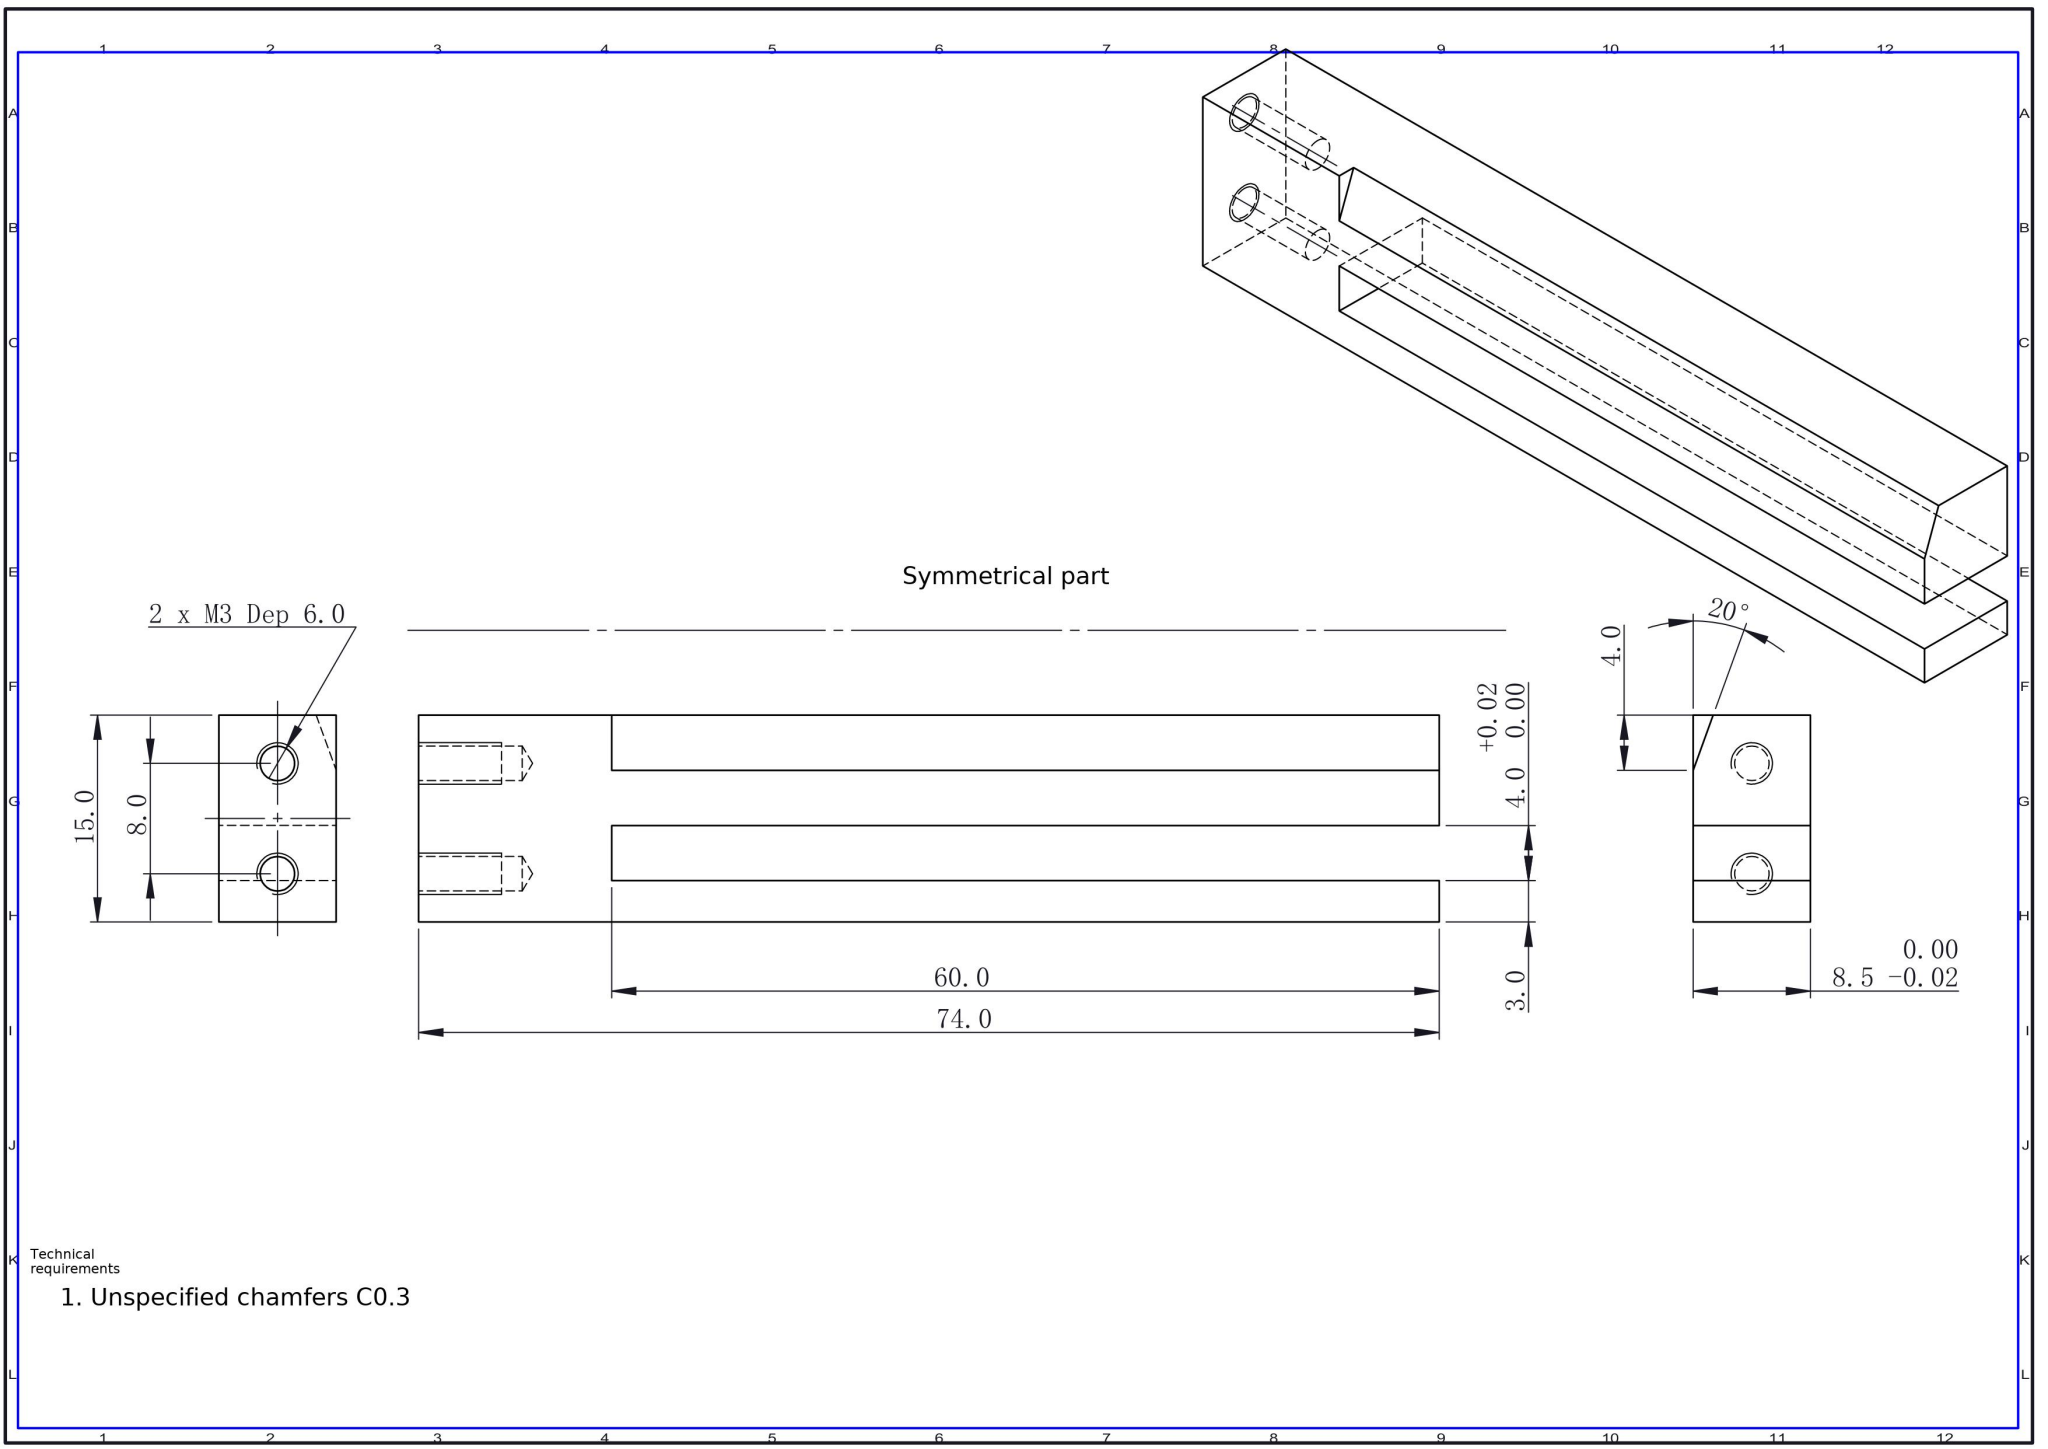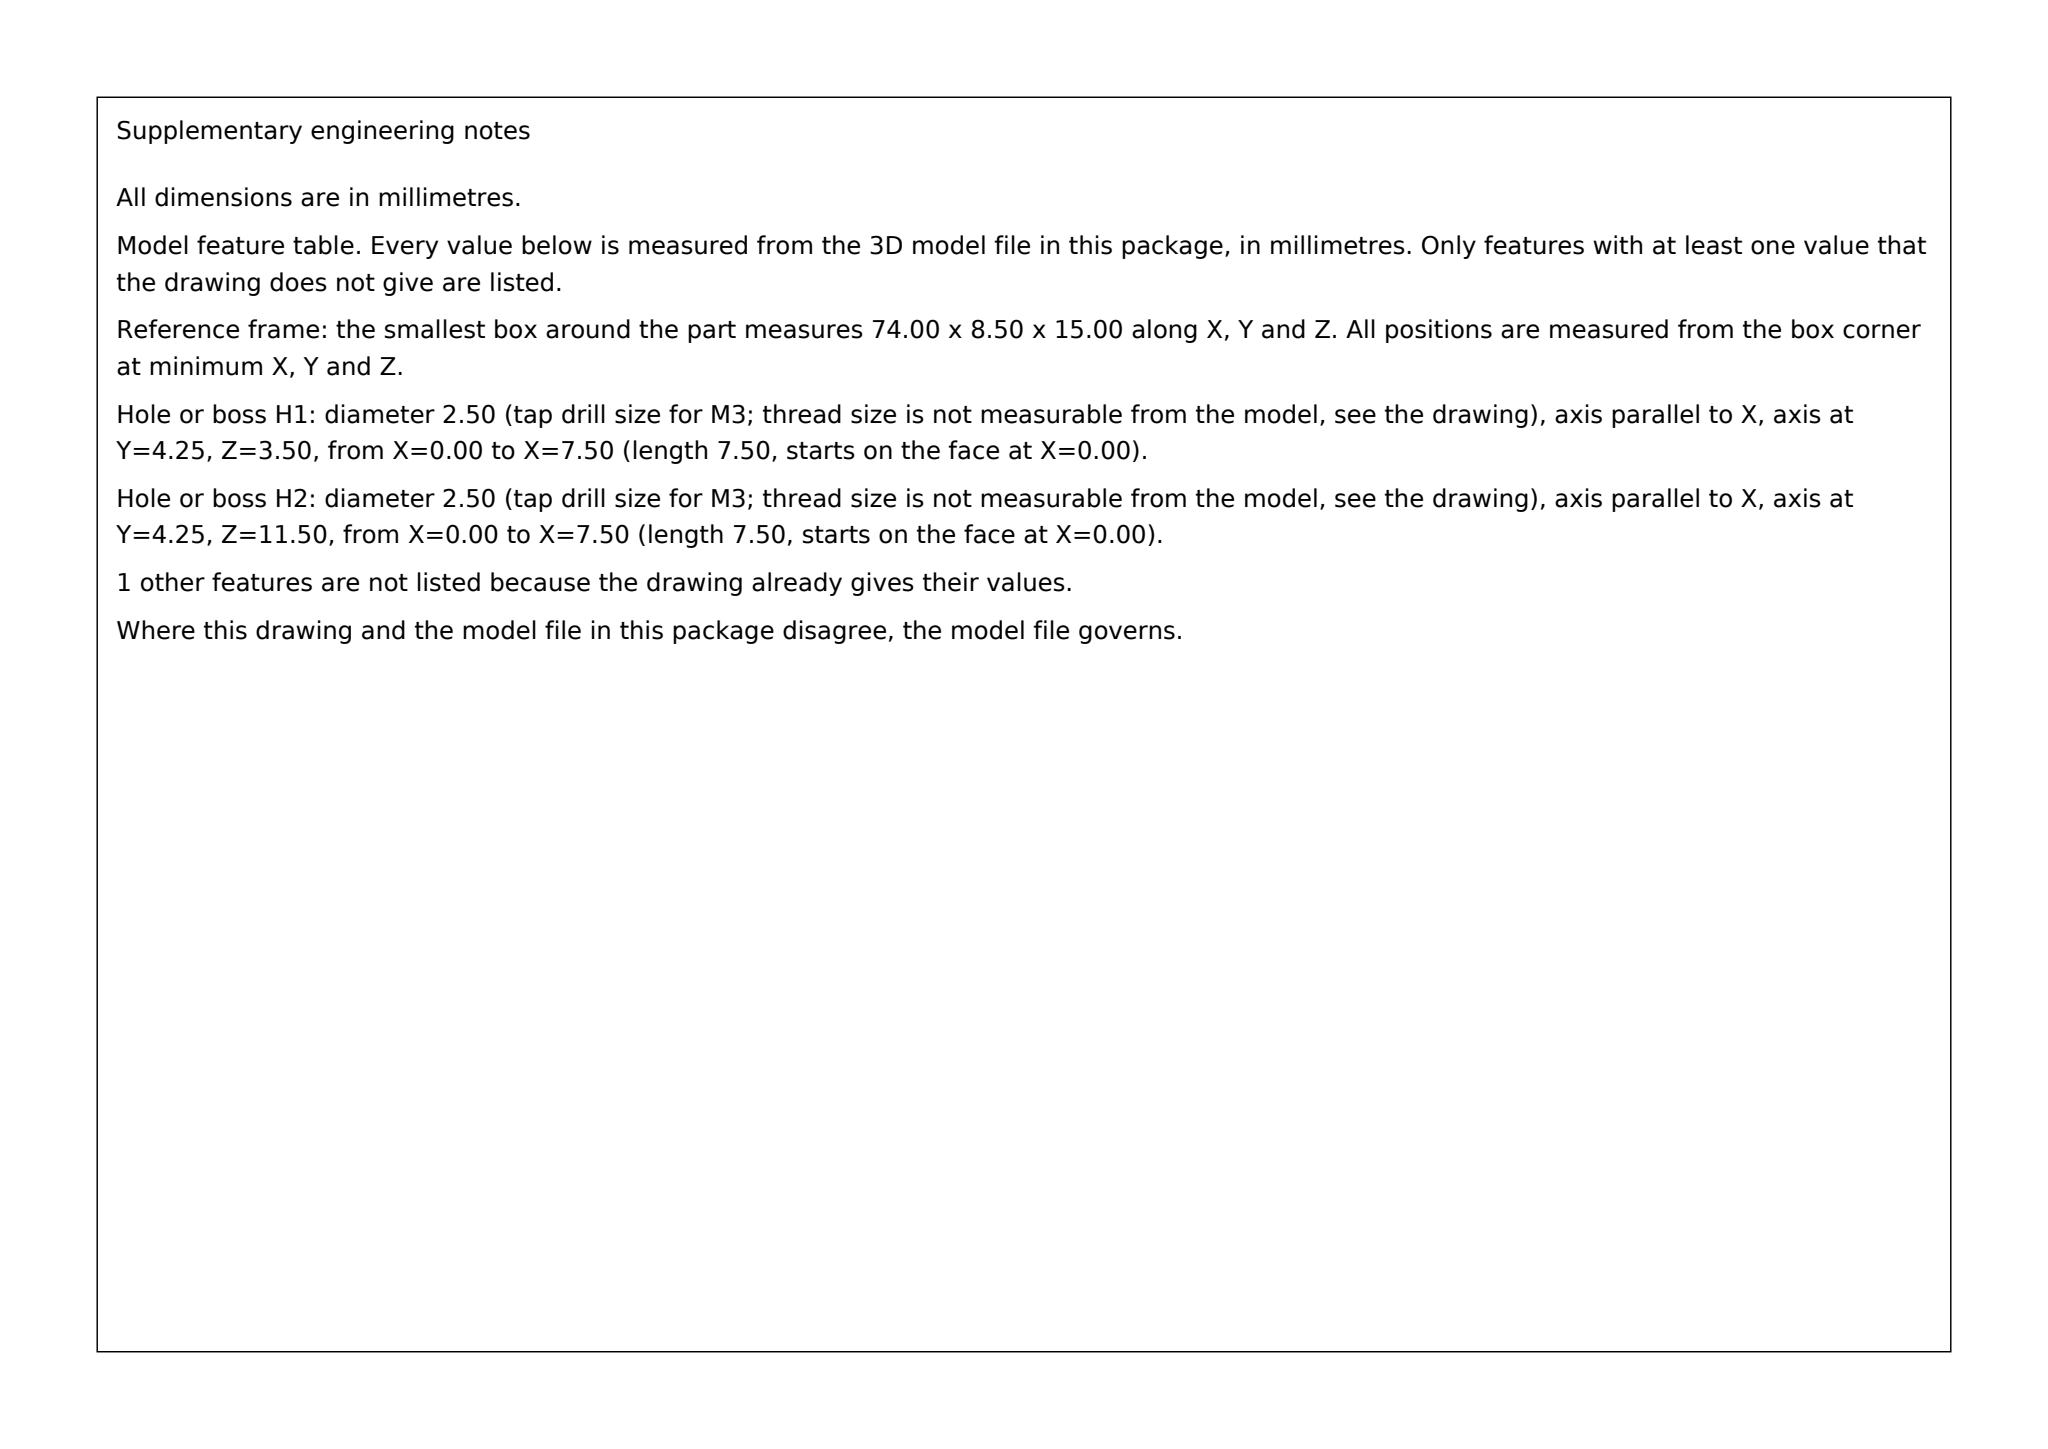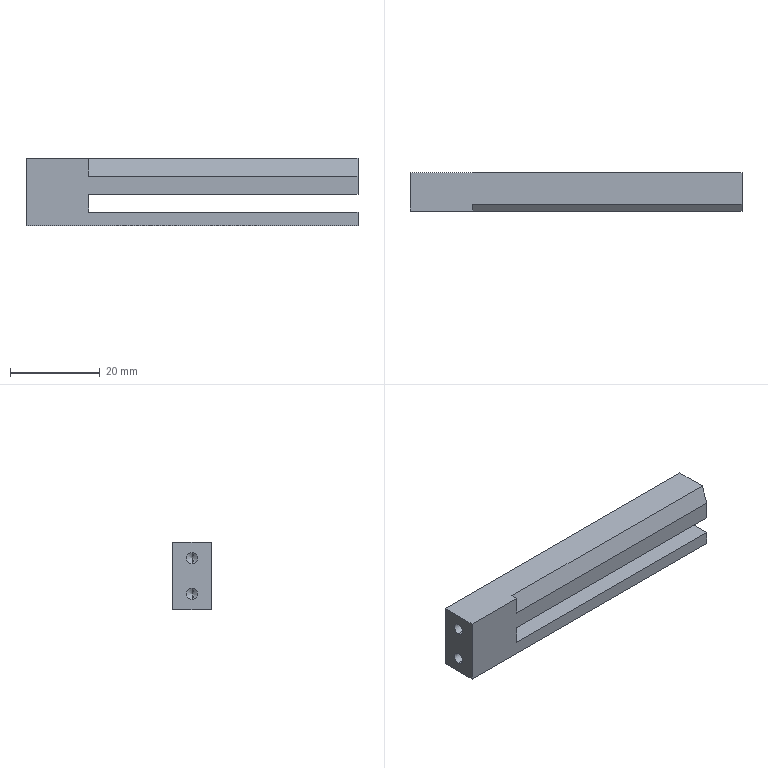Part | SolidWorks | mm | 1 solid | 20 faces | box 74 x 8.5 x 15 mm | volume 7144 mm3 | plane 12 | cylinder 4 | cone 4 | commonest cylinder face diameters 2.5 x4
build123d program:
from build123d import *

# Parameters (mm, degrees)
SKETCH1_W             = 74
SKETCH1_H             = 8.5
BOSS_EXTRUDE1_DEPTH   = 15
SKETCH4_W             = 60
SKETCH4_H             = 4
CUT_EXTRUDE1_DEPTH    = 76.982
M3_TAPPED_HOLE1_D     = 2.5
M3_TAPPED_HOLE1_DEPTH = 7.5
M3_TAPPED_HOLE1_TIP   = 0.7511
CUT_EXTRUDE2_DEPTH    = 60


with BuildPart() as part:
    # Sketch1 → Boss-Extrude1 (new body)
    with BuildSketch(Plane.XY):
        with Locations((37, 4.25)):
            Rectangle(SKETCH1_W, SKETCH1_H)
    extrude(amount=BOSS_EXTRUDE1_DEPTH)

    # Sketch4 → Cut-Extrude1 (cut, through all)
    with BuildSketch(Plane.XZ):
        with Locations((44, 5)):
            Rectangle(SKETCH4_W, SKETCH4_H)
    extrude(amount=-CUT_EXTRUDE1_DEPTH, mode=Mode.SUBTRACT)

    # M3 Tapped Hole1
    with Locations(Plane.ZY):
        with Locations((11.5, 4.25), (3.5, 4.25)):
            Hole(M3_TAPPED_HOLE1_D / 2, depth=M3_TAPPED_HOLE1_DEPTH)
            with Locations((0, 0, -(M3_TAPPED_HOLE1_DEPTH + M3_TAPPED_HOLE1_TIP / 2))):  # 118° drill point
                Cone(0, M3_TAPPED_HOLE1_D / 2, M3_TAPPED_HOLE1_TIP, mode=Mode.SUBTRACT)

    # Sketch7 → Cut-Extrude2 (cut)
    with BuildSketch(Plane(origin=(74, 0, 0), x_dir=(0, 0, -1), z_dir=(1, 0, 0))):
        Polygon((-15, 1.456), (-11, 0), (-15, 0), align=None)
    extrude(amount=-CUT_EXTRUDE2_DEPTH, mode=Mode.SUBTRACT)


solid = part.part
STEP:
#1=CARTESIAN_POINT('',(7.5,4.25,10.25));
#2=VERTEX_POINT('',#1);
#3=CARTESIAN_POINT('',(7.5,4.25,12.75));
#4=VERTEX_POINT('',#3);
#5=CARTESIAN_POINT('',(7.5,4.25,11.5));
#6=DIRECTION('',(-1.,0.,0.));
#7=DIRECTION('',(0.,0.,1.));
#8=AXIS2_PLACEMENT_3D('',#5,#6,#7);
#9=CIRCLE('',#8,1.25);
#10=EDGE_CURVE('',#2,#4,#9,.T.);
#11=ORIENTED_EDGE('',*,*,#10,.F.);
#12=CARTESIAN_POINT('',(-0.,4.25,10.25));
#13=VERTEX_POINT('',#12);
#14=CARTESIAN_POINT('',(0.,4.25,10.25));
#15=DIRECTION('',(-1.,0.,0.));
#16=VECTOR('',#15,1000.);
#17=LINE('',#14,#16);
#18=EDGE_CURVE('',#2,#13,#17,.T.);
#19=ORIENTED_EDGE('',*,*,#18,.T.);
#20=CARTESIAN_POINT('',(-0.,4.25,12.75));
#21=VERTEX_POINT('',#20);
#22=CARTESIAN_POINT('',(-0.,4.25,11.5));
#23=DIRECTION('',(-1.,0.,0.));
#24=DIRECTION('',(0.,0.,1.));
#25=AXIS2_PLACEMENT_3D('',#22,#23,#24);
#26=CIRCLE('',#25,1.25);
#27=EDGE_CURVE('',#13,#21,#26,.T.);
#28=ORIENTED_EDGE('',*,*,#27,.T.);
#29=CARTESIAN_POINT('',(0.,4.25,12.75));
#30=DIRECTION('',(-1.,0.,0.));
#31=VECTOR('',#30,1000.);
#32=LINE('',#29,#31);
#33=EDGE_CURVE('',#4,#21,#32,.T.);
#34=ORIENTED_EDGE('',*,*,#33,.F.);
#35=EDGE_LOOP('',(#11,#19,#28,#34));
#36=FACE_OUTER_BOUND('',#35,.T.);
#37=CARTESIAN_POINT('',(0.,4.25,11.5));
#38=DIRECTION('',(-1.,0.,0.));
#39=DIRECTION('',(0.,0.,1.));
#40=AXIS2_PLACEMENT_3D('',#37,#38,#39);
#41=CYLINDRICAL_SURFACE('',#40,1.25);
#42=ADVANCED_FACE('',(#36),#41,.F.);
#43=CARTESIAN_POINT('',(8.251,4.25,11.5));
#44=VERTEX_POINT('',#43);
#45=CARTESIAN_POINT('',(7.5,4.25,12.75));
#46=DIRECTION('',(-0.515,0.,0.8572));
#47=VECTOR('',#46,1000.);
#48=LINE('',#45,#47);
#49=EDGE_CURVE('',#44,#4,#48,.T.);
#50=ORIENTED_EDGE('',*,*,#49,.F.);
#51=CARTESIAN_POINT('',(7.5,4.25,10.25));
#52=DIRECTION('',(-0.515,0.,-0.8572));
#53=VECTOR('',#52,1000.);
#54=LINE('',#51,#53);
#55=EDGE_CURVE('',#44,#2,#54,.T.);
#56=ORIENTED_EDGE('',*,*,#55,.T.);
#57=ORIENTED_EDGE('',*,*,#10,.T.);
#58=EDGE_LOOP('',(#50,#56,#57));
#59=FACE_OUTER_BOUND('',#58,.T.);
#60=CARTESIAN_POINT('',(7.5,4.25,11.5));
#61=DIRECTION('',(-1.,0.,0.));
#62=DIRECTION('',(0.,0.,1.));
#63=AXIS2_PLACEMENT_3D('',#60,#61,#62);
#64=CONICAL_SURFACE('',#63,1.25,1.03);
#65=ADVANCED_FACE('',(#59),#64,.F.);
#66=CARTESIAN_POINT('',(7.5,4.25,2.25));
#67=VERTEX_POINT('',#66);
#68=CARTESIAN_POINT('',(7.5,4.25,4.75));
#69=VERTEX_POINT('',#68);
#70=CARTESIAN_POINT('',(7.5,4.25,3.5));
#71=DIRECTION('',(-1.,0.,0.));
#72=DIRECTION('',(0.,0.,1.));
#73=AXIS2_PLACEMENT_3D('',#70,#71,#72);
#74=CIRCLE('',#73,1.25);
#75=EDGE_CURVE('',#67,#69,#74,.T.);
#76=ORIENTED_EDGE('',*,*,#75,.F.);
#77=CARTESIAN_POINT('',(-0.,4.25,2.25));
#78=VERTEX_POINT('',#77);
#79=CARTESIAN_POINT('',(0.,4.25,2.25));
#80=DIRECTION('',(-1.,0.,0.));
#81=VECTOR('',#80,1000.);
#82=LINE('',#79,#81);
#83=EDGE_CURVE('',#67,#78,#82,.T.);
#84=ORIENTED_EDGE('',*,*,#83,.T.);
#85=CARTESIAN_POINT('',(-0.,4.25,4.75));
#86=VERTEX_POINT('',#85);
#87=CARTESIAN_POINT('',(-0.,4.25,3.5));
#88=DIRECTION('',(-1.,0.,0.));
#89=DIRECTION('',(0.,0.,1.));
#90=AXIS2_PLACEMENT_3D('',#87,#88,#89);
#91=CIRCLE('',#90,1.25);
#92=EDGE_CURVE('',#78,#86,#91,.T.);
#93=ORIENTED_EDGE('',*,*,#92,.T.);
#94=CARTESIAN_POINT('',(0.,4.25,4.75));
#95=DIRECTION('',(-1.,0.,0.));
#96=VECTOR('',#95,1000.);
#97=LINE('',#94,#96);
#98=EDGE_CURVE('',#69,#86,#97,.T.);
#99=ORIENTED_EDGE('',*,*,#98,.F.);
#100=EDGE_LOOP('',(#76,#84,#93,#99));
#101=FACE_OUTER_BOUND('',#100,.T.);
#102=CARTESIAN_POINT('',(0.,4.25,3.5));
#103=DIRECTION('',(-1.,0.,0.));
#104=DIRECTION('',(0.,0.,1.));
#105=AXIS2_PLACEMENT_3D('',#102,#103,#104);
#106=CYLINDRICAL_SURFACE('',#105,1.25);
#107=ADVANCED_FACE('',(#101),#106,.F.);
#108=CARTESIAN_POINT('',(8.251,4.25,3.5));
#109=VERTEX_POINT('',#108);
#110=CARTESIAN_POINT('',(7.5,4.25,4.75));
#111=DIRECTION('',(-0.515,0.,0.8572));
#112=VECTOR('',#111,1000.);
#113=LINE('',#110,#112);
#114=EDGE_CURVE('',#109,#69,#113,.T.);
#115=ORIENTED_EDGE('',*,*,#114,.F.);
#116=CARTESIAN_POINT('',(7.5,4.25,2.25));
#117=DIRECTION('',(-0.515,0.,-0.8572));
#118=VECTOR('',#117,1000.);
#119=LINE('',#116,#118);
#120=EDGE_CURVE('',#109,#67,#119,.T.);
#121=ORIENTED_EDGE('',*,*,#120,.T.);
#122=ORIENTED_EDGE('',*,*,#75,.T.);
#123=EDGE_LOOP('',(#115,#121,#122));
#124=FACE_OUTER_BOUND('',#123,.T.);
#125=CARTESIAN_POINT('',(7.5,4.25,3.5));
#126=DIRECTION('',(-1.,0.,0.));
#127=DIRECTION('',(0.,0.,1.));
#128=AXIS2_PLACEMENT_3D('',#125,#126,#127);
#129=CONICAL_SURFACE('',#128,1.25,1.03);
#130=ADVANCED_FACE('',(#124),#129,.F.);
#131=CARTESIAN_POINT('',(74.,8.5,3.));
#132=VERTEX_POINT('',#131);
#133=CARTESIAN_POINT('',(74.,8.5,0.));
#134=VERTEX_POINT('',#133);
#135=CARTESIAN_POINT('',(74.,8.5,15.));
#136=DIRECTION('',(0.,0.,-1.));
#137=VECTOR('',#136,1000.);
#138=LINE('',#135,#137);
#139=EDGE_CURVE('',#132,#134,#138,.T.);
#140=ORIENTED_EDGE('',*,*,#139,.F.);
#141=CARTESIAN_POINT('',(74.,0.,3.));
#142=VERTEX_POINT('',#141);
#143=CARTESIAN_POINT('',(74.,8.5,3.));
#144=DIRECTION('',(0.,-1.,0.));
#145=VECTOR('',#144,1000.);
#146=LINE('',#143,#145);
#147=EDGE_CURVE('',#132,#142,#146,.T.);
#148=ORIENTED_EDGE('',*,*,#147,.T.);
#149=CARTESIAN_POINT('',(74.,0.,0.));
#150=VERTEX_POINT('',#149);
#151=CARTESIAN_POINT('',(74.,0.,15.));
#152=DIRECTION('',(0.,0.,-1.));
#153=VECTOR('',#152,1000.);
#154=LINE('',#151,#153);
#155=EDGE_CURVE('',#142,#150,#154,.T.);
#156=ORIENTED_EDGE('',*,*,#155,.T.);
#157=CARTESIAN_POINT('',(74.,0.,0.));
#158=DIRECTION('',(0.,1.,0.));
#159=VECTOR('',#158,1000.);
#160=LINE('',#157,#159);
#161=EDGE_CURVE('',#150,#134,#160,.T.);
#162=ORIENTED_EDGE('',*,*,#161,.T.);
#163=EDGE_LOOP('',(#140,#148,#156,#162));
#164=FACE_OUTER_BOUND('',#163,.T.);
#165=CARTESIAN_POINT('',(74.,0.,15.));
#166=DIRECTION('',(-1.,0.,0.));
#167=DIRECTION('',(0.,0.,1.));
#168=AXIS2_PLACEMENT_3D('',#165,#166,#167);
#169=PLANE('',#168);
#170=ADVANCED_FACE('',(#164),#169,.F.);
#171=CARTESIAN_POINT('',(-0.,4.25,11.5));
#172=DIRECTION('',(-1.,0.,0.));
#173=DIRECTION('',(0.,0.,1.));
#174=AXIS2_PLACEMENT_3D('',#171,#172,#173);
#175=CIRCLE('',#174,1.25);
#176=EDGE_CURVE('',#21,#13,#175,.T.);
#177=ORIENTED_EDGE('',*,*,#176,.F.);
#178=ORIENTED_EDGE('',*,*,#27,.F.);
#179=EDGE_LOOP('',(#177,#178));
#180=FACE_BOUND('',#179,.T.);
#181=CARTESIAN_POINT('',(-0.,4.25,3.5));
#182=DIRECTION('',(-1.,0.,0.));
#183=DIRECTION('',(0.,0.,1.));
#184=AXIS2_PLACEMENT_3D('',#181,#182,#183);
#185=CIRCLE('',#184,1.25);
#186=EDGE_CURVE('',#86,#78,#185,.T.);
#187=ORIENTED_EDGE('',*,*,#186,.F.);
#188=ORIENTED_EDGE('',*,*,#92,.F.);
#189=EDGE_LOOP('',(#187,#188));
#190=FACE_BOUND('',#189,.T.);
#191=CARTESIAN_POINT('',(0.,8.5,0.));
#192=VERTEX_POINT('',#191);
#193=CARTESIAN_POINT('',(0.,0.,0.));
#194=VERTEX_POINT('',#193);
#195=CARTESIAN_POINT('',(0.,0.,0.));
#196=DIRECTION('',(0.,-1.,0.));
#197=VECTOR('',#196,1000.);
#198=LINE('',#195,#197);
#199=EDGE_CURVE('',#192,#194,#198,.T.);
#200=ORIENTED_EDGE('',*,*,#199,.T.);
#201=CARTESIAN_POINT('',(0.,0.,15.));
#202=VERTEX_POINT('',#201);
#203=CARTESIAN_POINT('',(0.,0.,15.));
#204=DIRECTION('',(0.,0.,-1.));
#205=VECTOR('',#204,1000.);
#206=LINE('',#203,#205);
#207=EDGE_CURVE('',#202,#194,#206,.T.);
#208=ORIENTED_EDGE('',*,*,#207,.F.);
#209=CARTESIAN_POINT('',(0.,8.5,15.));
#210=VERTEX_POINT('',#209);
#211=CARTESIAN_POINT('',(0.,0.,15.));
#212=DIRECTION('',(0.,-1.,0.));
#213=VECTOR('',#212,1000.);
#214=LINE('',#211,#213);
#215=EDGE_CURVE('',#210,#202,#214,.T.);
#216=ORIENTED_EDGE('',*,*,#215,.F.);
#217=CARTESIAN_POINT('',(0.,8.5,15.));
#218=DIRECTION('',(0.,0.,-1.));
#219=VECTOR('',#218,1000.);
#220=LINE('',#217,#219);
#221=EDGE_CURVE('',#210,#192,#220,.T.);
#222=ORIENTED_EDGE('',*,*,#221,.T.);
#223=EDGE_LOOP('',(#200,#208,#216,#222));
#224=FACE_OUTER_BOUND('',#223,.T.);
#225=CARTESIAN_POINT('',(0.,0.,15.));
#226=DIRECTION('',(1.,0.,0.));
#227=DIRECTION('',(0.,0.,-1.));
#228=AXIS2_PLACEMENT_3D('',#225,#226,#227);
#229=PLANE('',#228);
#230=ADVANCED_FACE('',(#180,#190,#224),#229,.F.);
#231=CARTESIAN_POINT('',(74.,0.,11.));
#232=VERTEX_POINT('',#231);
#233=CARTESIAN_POINT('',(74.,0.,7.));
#234=VERTEX_POINT('',#233);
#235=CARTESIAN_POINT('',(74.,0.,15.));
#236=DIRECTION('',(0.,0.,-1.));
#237=VECTOR('',#236,1000.);
#238=LINE('',#235,#237);
#239=EDGE_CURVE('',#232,#234,#238,.T.);
#240=ORIENTED_EDGE('',*,*,#239,.F.);
#241=CARTESIAN_POINT('',(14.,0.,11.));
#242=VERTEX_POINT('',#241);
#243=CARTESIAN_POINT('',(14.,0.,11.));
#244=DIRECTION('',(1.,0.,0.));
#245=VECTOR('',#244,1000.);
#246=LINE('',#243,#245);
#247=EDGE_CURVE('',#242,#232,#246,.T.);
#248=ORIENTED_EDGE('',*,*,#247,.F.);
#249=CARTESIAN_POINT('',(14.,0.,15.));
#250=VERTEX_POINT('',#249);
#251=CARTESIAN_POINT('',(14.,0.,11.));
#252=DIRECTION('',(0.,0.,-1.));
#253=VECTOR('',#252,1000.);
#254=LINE('',#251,#253);
#255=EDGE_CURVE('',#250,#242,#254,.T.);
#256=ORIENTED_EDGE('',*,*,#255,.F.);
#257=CARTESIAN_POINT('',(0.,0.,15.));
#258=DIRECTION('',(1.,0.,0.));
#259=VECTOR('',#258,1000.);
#260=LINE('',#257,#259);
#261=EDGE_CURVE('',#202,#250,#260,.T.);
#262=ORIENTED_EDGE('',*,*,#261,.F.);
#263=ORIENTED_EDGE('',*,*,#207,.T.);
#264=CARTESIAN_POINT('',(0.,0.,0.));
#265=DIRECTION('',(1.,0.,0.));
#266=VECTOR('',#265,1000.);
#267=LINE('',#264,#266);
#268=EDGE_CURVE('',#194,#150,#267,.T.);
#269=ORIENTED_EDGE('',*,*,#268,.T.);
#270=ORIENTED_EDGE('',*,*,#155,.F.);
#271=CARTESIAN_POINT('',(14.,0.,3.));
#272=VERTEX_POINT('',#271);
#273=CARTESIAN_POINT('',(74.,0.,3.));
#274=DIRECTION('',(1.,0.,0.));
#275=VECTOR('',#274,1000.);
#276=LINE('',#273,#275);
#277=EDGE_CURVE('',#272,#142,#276,.T.);
#278=ORIENTED_EDGE('',*,*,#277,.F.);
#279=CARTESIAN_POINT('',(14.,0.,7.));
#280=VERTEX_POINT('',#279);
#281=CARTESIAN_POINT('',(14.,0.,7.));
#282=DIRECTION('',(0.,0.,-1.));
#283=VECTOR('',#282,1000.);
#284=LINE('',#281,#283);
#285=EDGE_CURVE('',#280,#272,#284,.T.);
#286=ORIENTED_EDGE('',*,*,#285,.F.);
#287=CARTESIAN_POINT('',(74.,0.,7.));
#288=DIRECTION('',(-1.,0.,-0.));
#289=VECTOR('',#288,1000.);
#290=LINE('',#287,#289);
#291=EDGE_CURVE('',#234,#280,#290,.T.);
#292=ORIENTED_EDGE('',*,*,#291,.F.);
#293=EDGE_LOOP('',(#240,#248,#256,#262,#263,#269,#270,#278,#286,#292));
#294=FACE_OUTER_BOUND('',#293,.T.);
#295=CARTESIAN_POINT('',(0.,0.,15.));
#296=DIRECTION('',(0.,1.,0.));
#297=DIRECTION('',(0.,0.,1.));
#298=AXIS2_PLACEMENT_3D('',#295,#296,#297);
#299=PLANE('',#298);
#300=ADVANCED_FACE('',(#294),#299,.F.);
#301=CARTESIAN_POINT('',(74.,1.456,15.));
#302=VERTEX_POINT('',#301);
#303=CARTESIAN_POINT('',(74.,8.5,15.));
#304=VERTEX_POINT('',#303);
#305=CARTESIAN_POINT('',(74.,0.,15.));
#306=DIRECTION('',(0.,1.,0.));
#307=VECTOR('',#306,1000.);
#308=LINE('',#305,#307);
#309=EDGE_CURVE('',#302,#304,#308,.T.);
#310=ORIENTED_EDGE('',*,*,#309,.F.);
#311=CARTESIAN_POINT('',(74.,1.456,15.));
#312=DIRECTION('',(0.,0.342,0.9397));
#313=VECTOR('',#312,1000.);
#314=LINE('',#311,#313);
#315=EDGE_CURVE('',#232,#302,#314,.T.);
#316=ORIENTED_EDGE('',*,*,#315,.F.);
#317=ORIENTED_EDGE('',*,*,#239,.T.);
#318=CARTESIAN_POINT('',(74.,8.5,7.));
#319=VERTEX_POINT('',#318);
#320=CARTESIAN_POINT('',(74.,8.5,7.));
#321=DIRECTION('',(0.,-1.,0.));
#322=VECTOR('',#321,1000.);
#323=LINE('',#320,#322);
#324=EDGE_CURVE('',#319,#234,#323,.T.);
#325=ORIENTED_EDGE('',*,*,#324,.F.);
#326=CARTESIAN_POINT('',(74.,8.5,15.));
#327=DIRECTION('',(0.,0.,-1.));
#328=VECTOR('',#327,1000.);
#329=LINE('',#326,#328);
#330=EDGE_CURVE('',#304,#319,#329,.T.);
#331=ORIENTED_EDGE('',*,*,#330,.F.);
#332=EDGE_LOOP('',(#310,#316,#317,#325,#331));
#333=FACE_OUTER_BOUND('',#332,.T.);
#334=CARTESIAN_POINT('',(74.,0.,15.));
#335=DIRECTION('',(-1.,0.,0.));
#336=DIRECTION('',(0.,0.,1.));
#337=AXIS2_PLACEMENT_3D('',#334,#335,#336);
#338=PLANE('',#337);
#339=ADVANCED_FACE('',(#333),#338,.F.);
#340=CARTESIAN_POINT('',(14.,8.5,7.));
#341=VERTEX_POINT('',#340);
#342=CARTESIAN_POINT('',(14.,8.5,3.));
#343=VERTEX_POINT('',#342);
#344=CARTESIAN_POINT('',(14.,8.5,7.));
#345=DIRECTION('',(0.,0.,-1.));
#346=VECTOR('',#345,1000.);
#347=LINE('',#344,#346);
#348=EDGE_CURVE('',#341,#343,#347,.T.);
#349=ORIENTED_EDGE('',*,*,#348,.T.);
#350=CARTESIAN_POINT('',(74.,8.5,3.));
#351=DIRECTION('',(1.,0.,0.));
#352=VECTOR('',#351,1000.);
#353=LINE('',#350,#352);
#354=EDGE_CURVE('',#343,#132,#353,.T.);
#355=ORIENTED_EDGE('',*,*,#354,.T.);
#356=ORIENTED_EDGE('',*,*,#139,.T.);
#357=CARTESIAN_POINT('',(0.,8.5,0.));
#358=DIRECTION('',(-1.,0.,0.));
#359=VECTOR('',#358,1000.);
#360=LINE('',#357,#359);
#361=EDGE_CURVE('',#134,#192,#360,.T.);
#362=ORIENTED_EDGE('',*,*,#361,.T.);
#363=ORIENTED_EDGE('',*,*,#221,.F.);
#364=CARTESIAN_POINT('',(0.,8.5,15.));
#365=DIRECTION('',(-1.,0.,0.));
#366=VECTOR('',#365,1000.);
#367=LINE('',#364,#366);
#368=EDGE_CURVE('',#304,#210,#367,.T.);
#369=ORIENTED_EDGE('',*,*,#368,.F.);
#370=ORIENTED_EDGE('',*,*,#330,.T.);
#371=CARTESIAN_POINT('',(74.,8.5,7.));
#372=DIRECTION('',(-1.,0.,-0.));
#373=VECTOR('',#372,1000.);
#374=LINE('',#371,#373);
#375=EDGE_CURVE('',#319,#341,#374,.T.);
#376=ORIENTED_EDGE('',*,*,#375,.T.);
#377=EDGE_LOOP('',(#349,#355,#356,#362,#363,#369,#370,#376));
#378=FACE_OUTER_BOUND('',#377,.T.);
#379=CARTESIAN_POINT('',(0.,8.5,15.));
#380=DIRECTION('',(0.,-1.,0.));
#381=DIRECTION('',(0.,0.,-1.));
#382=AXIS2_PLACEMENT_3D('',#379,#380,#381);
#383=PLANE('',#382);
#384=ADVANCED_FACE('',(#378),#383,.F.);
#385=CARTESIAN_POINT('',(14.,1.456,15.));
#386=VERTEX_POINT('',#385);
#387=CARTESIAN_POINT('',(14.,0.,15.));
#388=DIRECTION('',(0.,-1.,-0.));
#389=VECTOR('',#388,1000.);
#390=LINE('',#387,#389);
#391=EDGE_CURVE('',#386,#250,#390,.T.);
#392=ORIENTED_EDGE('',*,*,#391,.F.);
#393=CARTESIAN_POINT('',(14.,1.456,15.));
#394=DIRECTION('',(1.,0.,0.));
#395=VECTOR('',#394,1000.);
#396=LINE('',#393,#395);
#397=EDGE_CURVE('',#386,#302,#396,.T.);
#398=ORIENTED_EDGE('',*,*,#397,.T.);
#399=ORIENTED_EDGE('',*,*,#309,.T.);
#400=ORIENTED_EDGE('',*,*,#368,.T.);
#401=ORIENTED_EDGE('',*,*,#215,.T.);
#402=ORIENTED_EDGE('',*,*,#261,.T.);
#403=EDGE_LOOP('',(#392,#398,#399,#400,#401,#402));
#404=FACE_OUTER_BOUND('',#403,.T.);
#405=CARTESIAN_POINT('',(0.,0.,15.));
#406=DIRECTION('',(0.,0.,-1.));
#407=DIRECTION('',(-1.,0.,0.));
#408=AXIS2_PLACEMENT_3D('',#405,#406,#407);
#409=PLANE('',#408);
#410=ADVANCED_FACE('',(#404),#409,.F.);
#411=ORIENTED_EDGE('',*,*,#199,.F.);
#412=ORIENTED_EDGE('',*,*,#361,.F.);
#413=ORIENTED_EDGE('',*,*,#161,.F.);
#414=ORIENTED_EDGE('',*,*,#268,.F.);
#415=EDGE_LOOP('',(#411,#412,#413,#414));
#416=FACE_OUTER_BOUND('',#415,.T.);
#417=CARTESIAN_POINT('',(0.,0.,0.));
#418=DIRECTION('',(0.,0.,-1.));
#419=DIRECTION('',(-1.,0.,0.));
#420=AXIS2_PLACEMENT_3D('',#417,#418,#419);
#421=PLANE('',#420);
#422=ADVANCED_FACE('',(#416),#421,.T.);
#423=ORIENTED_EDGE('',*,*,#277,.T.);
#424=ORIENTED_EDGE('',*,*,#147,.F.);
#425=ORIENTED_EDGE('',*,*,#354,.F.);
#426=CARTESIAN_POINT('',(14.,8.5,3.));
#427=DIRECTION('',(0.,-1.,0.));
#428=VECTOR('',#427,1000.);
#429=LINE('',#426,#428);
#430=EDGE_CURVE('',#343,#272,#429,.T.);
#431=ORIENTED_EDGE('',*,*,#430,.T.);
#432=EDGE_LOOP('',(#423,#424,#425,#431));
#433=FACE_OUTER_BOUND('',#432,.T.);
#434=CARTESIAN_POINT('',(74.,8.5,3.));
#435=DIRECTION('',(0.,0.,-1.));
#436=DIRECTION('',(-1.,0.,-0.));
#437=AXIS2_PLACEMENT_3D('',#434,#435,#436);
#438=PLANE('',#437);
#439=ADVANCED_FACE('',(#433),#438,.F.);
#440=ORIENTED_EDGE('',*,*,#285,.T.);
#441=ORIENTED_EDGE('',*,*,#430,.F.);
#442=ORIENTED_EDGE('',*,*,#348,.F.);
#443=CARTESIAN_POINT('',(14.,8.5,7.));
#444=DIRECTION('',(0.,-1.,0.));
#445=VECTOR('',#444,1000.);
#446=LINE('',#443,#445);
#447=EDGE_CURVE('',#341,#280,#446,.T.);
#448=ORIENTED_EDGE('',*,*,#447,.T.);
#449=EDGE_LOOP('',(#440,#441,#442,#448));
#450=FACE_OUTER_BOUND('',#449,.T.);
#451=CARTESIAN_POINT('',(14.,8.5,7.));
#452=DIRECTION('',(-1.,0.,0.));
#453=DIRECTION('',(0.,0.,1.));
#454=AXIS2_PLACEMENT_3D('',#451,#452,#453);
#455=PLANE('',#454);
#456=ADVANCED_FACE('',(#450),#455,.F.);
#457=ORIENTED_EDGE('',*,*,#291,.T.);
#458=ORIENTED_EDGE('',*,*,#447,.F.);
#459=ORIENTED_EDGE('',*,*,#375,.F.);
#460=ORIENTED_EDGE('',*,*,#324,.T.);
#461=EDGE_LOOP('',(#457,#458,#459,#460));
#462=FACE_OUTER_BOUND('',#461,.T.);
#463=CARTESIAN_POINT('',(74.,8.5,7.));
#464=DIRECTION('',(-0.,0.,1.));
#465=DIRECTION('',(1.,0.,0.));
#466=AXIS2_PLACEMENT_3D('',#463,#464,#465);
#467=PLANE('',#466);
#468=ADVANCED_FACE('',(#462),#467,.F.);
#469=ORIENTED_EDGE('',*,*,#120,.F.);
#470=ORIENTED_EDGE('',*,*,#114,.T.);
#471=CARTESIAN_POINT('',(7.5,4.25,3.5));
#472=DIRECTION('',(-1.,0.,0.));
#473=DIRECTION('',(0.,0.,1.));
#474=AXIS2_PLACEMENT_3D('',#471,#472,#473);
#475=CIRCLE('',#474,1.25);
#476=EDGE_CURVE('',#69,#67,#475,.T.);
#477=ORIENTED_EDGE('',*,*,#476,.T.);
#478=EDGE_LOOP('',(#469,#470,#477));
#479=FACE_OUTER_BOUND('',#478,.T.);
#480=CARTESIAN_POINT('',(7.5,4.25,3.5));
#481=DIRECTION('',(-1.,0.,0.));
#482=DIRECTION('',(0.,0.,1.));
#483=AXIS2_PLACEMENT_3D('',#480,#481,#482);
#484=CONICAL_SURFACE('',#483,1.25,1.03);
#485=ADVANCED_FACE('',(#479),#484,.F.);
#486=ORIENTED_EDGE('',*,*,#83,.F.);
#487=ORIENTED_EDGE('',*,*,#476,.F.);
#488=ORIENTED_EDGE('',*,*,#98,.T.);
#489=ORIENTED_EDGE('',*,*,#186,.T.);
#490=EDGE_LOOP('',(#486,#487,#488,#489));
#491=FACE_OUTER_BOUND('',#490,.T.);
#492=CARTESIAN_POINT('',(0.,4.25,3.5));
#493=DIRECTION('',(-1.,0.,0.));
#494=DIRECTION('',(0.,0.,1.));
#495=AXIS2_PLACEMENT_3D('',#492,#493,#494);
#496=CYLINDRICAL_SURFACE('',#495,1.25);
#497=ADVANCED_FACE('',(#491),#496,.F.);
#498=ORIENTED_EDGE('',*,*,#55,.F.);
#499=ORIENTED_EDGE('',*,*,#49,.T.);
#500=CARTESIAN_POINT('',(7.5,4.25,11.5));
#501=DIRECTION('',(-1.,0.,0.));
#502=DIRECTION('',(0.,0.,1.));
#503=AXIS2_PLACEMENT_3D('',#500,#501,#502);
#504=CIRCLE('',#503,1.25);
#505=EDGE_CURVE('',#4,#2,#504,.T.);
#506=ORIENTED_EDGE('',*,*,#505,.T.);
#507=EDGE_LOOP('',(#498,#499,#506));
#508=FACE_OUTER_BOUND('',#507,.T.);
#509=CARTESIAN_POINT('',(7.5,4.25,11.5));
#510=DIRECTION('',(-1.,0.,0.));
#511=DIRECTION('',(0.,0.,1.));
#512=AXIS2_PLACEMENT_3D('',#509,#510,#511);
#513=CONICAL_SURFACE('',#512,1.25,1.03);
#514=ADVANCED_FACE('',(#508),#513,.F.);
#515=ORIENTED_EDGE('',*,*,#18,.F.);
#516=ORIENTED_EDGE('',*,*,#505,.F.);
#517=ORIENTED_EDGE('',*,*,#33,.T.);
#518=ORIENTED_EDGE('',*,*,#176,.T.);
#519=EDGE_LOOP('',(#515,#516,#517,#518));
#520=FACE_OUTER_BOUND('',#519,.T.);
#521=CARTESIAN_POINT('',(0.,4.25,11.5));
#522=DIRECTION('',(-1.,0.,0.));
#523=DIRECTION('',(0.,0.,1.));
#524=AXIS2_PLACEMENT_3D('',#521,#522,#523);
#525=CYLINDRICAL_SURFACE('',#524,1.25);
#526=ADVANCED_FACE('',(#520),#525,.F.);
#527=ORIENTED_EDGE('',*,*,#315,.T.);
#528=ORIENTED_EDGE('',*,*,#397,.F.);
#529=CARTESIAN_POINT('',(14.,1.456,15.));
#530=DIRECTION('',(0.,0.342,0.9397));
#531=VECTOR('',#530,1000.);
#532=LINE('',#529,#531);
#533=EDGE_CURVE('',#242,#386,#532,.T.);
#534=ORIENTED_EDGE('',*,*,#533,.F.);
#535=ORIENTED_EDGE('',*,*,#247,.T.);
#536=EDGE_LOOP('',(#527,#528,#534,#535));
#537=FACE_OUTER_BOUND('',#536,.T.);
#538=CARTESIAN_POINT('',(14.,1.456,15.));
#539=DIRECTION('',(0.,0.9397,-0.342));
#540=DIRECTION('',(0.,0.342,0.9397));
#541=AXIS2_PLACEMENT_3D('',#538,#539,#540);
#542=PLANE('',#541);
#543=ADVANCED_FACE('',(#537),#542,.F.);
#544=ORIENTED_EDGE('',*,*,#391,.T.);
#545=ORIENTED_EDGE('',*,*,#255,.T.);
#546=ORIENTED_EDGE('',*,*,#533,.T.);
#547=EDGE_LOOP('',(#544,#545,#546));
#548=FACE_OUTER_BOUND('',#547,.T.);
#549=CARTESIAN_POINT('',(14.,0.,0.));
#550=DIRECTION('',(1.,0.,0.));
#551=DIRECTION('',(0.,0.,-1.));
#552=AXIS2_PLACEMENT_3D('',#549,#550,#551);
#553=PLANE('',#552);
#554=ADVANCED_FACE('',(#548),#553,.T.);
#555=CLOSED_SHELL('',(#42,#65,#107,#130,#170,#230,#300,#339,#384,#410,#422,#439,#456,#468,#485,#497,#514,#526,#543,#554));
#556=MANIFOLD_SOLID_BREP('',#555);
#557=CARTESIAN_POINT('',(0.,0.,0.));
#558=DIRECTION('',(0.,0.,1.));
#559=DIRECTION('',(1.,0.,0.));
#560=AXIS2_PLACEMENT_3D('',#557,#558,#559);
#561=(LENGTH_UNIT()NAMED_UNIT(*)SI_UNIT(.MILLI.,.METRE.));
#562=UNCERTAINTY_MEASURE_WITH_UNIT(LENGTH_MEASURE(0.00001),#561,'','');
#563=(NAMED_UNIT(*)PLANE_ANGLE_UNIT()SI_UNIT($,.RADIAN.));
#564=(NAMED_UNIT(*)SI_UNIT($,.STERADIAN.)SOLID_ANGLE_UNIT());
#565=(GEOMETRIC_REPRESENTATION_CONTEXT(3)GLOBAL_UNCERTAINTY_ASSIGNED_CONTEXT((#562))GLOBAL_UNIT_ASSIGNED_CONTEXT((#561,#563,#564))REPRESENTATION_CONTEXT('',''));
#566=ADVANCED_BREP_SHAPE_REPRESENTATION('',(#556,#560),#565);